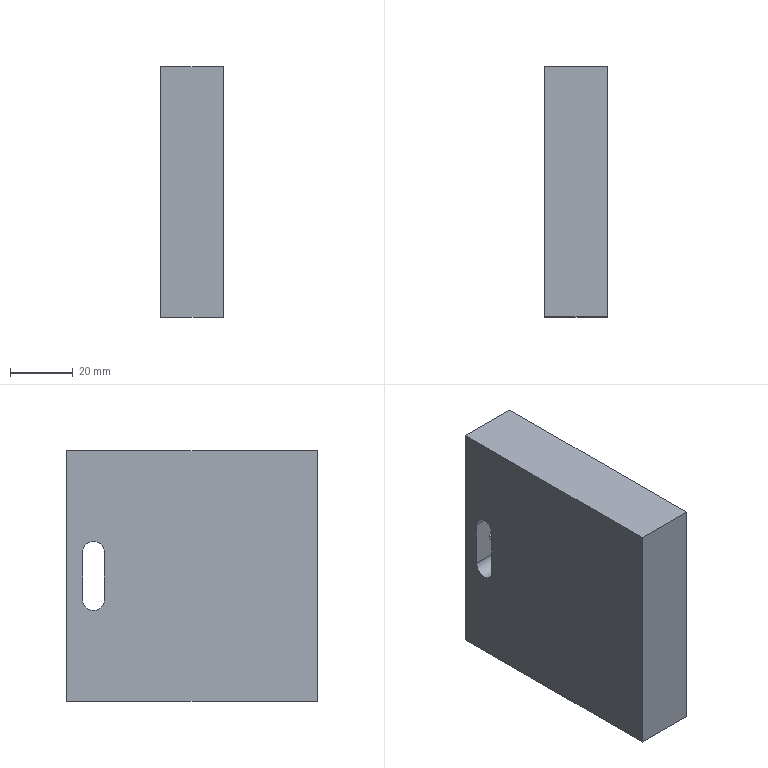Component | SolidWorks | LocatingDie-2_Die-1 | 1 solid | 14 faces | box 20 x 80 x 80 mm | volume 124605 mm3 | plane 10 | cylinder 4 | commonest cylinder face diameters 7 x3 8 x1
build123d program:
from build123d import *

# Parameters (mm, degrees)
SKETCH1_W      = 80
SKETCH1_H      = 80
EXTRUDE1_DEPTH = 20
EXTRUDE2_REACH = 95.62


with BuildPart() as part:
    # Sketch1 → Extrude1 (new body)
    with BuildSketch(Plane.XY):
        with Locations((-4.325, -1.62)):
            Rectangle(SKETCH1_W, SKETCH1_H)
        with BuildLine():
            Line((-11.825, 33.38), (3.175, 33.38))
            ThreePointArc((3.175, 33.38), (6.675, 29.88), (3.175, 26.38))
            Line((3.175, 26.38), (-11.825, 26.38))
            ThreePointArc((-11.825, 26.38), (-15.325, 29.88), (-11.825, 33.38))
        make_face(mode=Mode.SUBTRACT)
    extrude(amount=EXTRUDE1_DEPTH)

    # Sketch2 → Extrude2 (cut, up to next)
    with BuildSketch(Plane(origin=(0, 38.38, 0), x_dir=(1, 0, 0), z_dir=(0, 1, 0)), mode=Mode.PRIVATE) as extrude2_sk1:
        with BuildLine():
            Line((-0.3255, -20), (-8.325, -20))
            Line((-8.325, -20), (-8.325, -10))
            ThreePointArc((-8.325, -10), (-4.325, -6), (-0.3255, -10))
            Line((-0.3255, -10), (-0.3255, -20))
        make_face()
    extrude2_tool1 = extrude(extrude2_sk1.sketch, amount=-EXTRUDE2_REACH, mode=Mode.PRIVATE) & part.part
    add(extrude2_tool1.solids().sort_by_distance((-4.325, 38.38, 13.399))[0], mode=Mode.SUBTRACT)


solid = part.part

# Placed as in the assembly
solid = solid.moved(Location((-306.784, 563.808, 9.675), (0, 90, 0)))
STEP:
#1=COLOUR_RGB('',0.7922,0.8196,0.9333);
#2=FILL_AREA_STYLE_COLOUR('',#1);
#3=FILL_AREA_STYLE('',(#2));
#4=SURFACE_STYLE_FILL_AREA(#3);
#5=SURFACE_SIDE_STYLE('',(#4));
#6=SURFACE_STYLE_USAGE(.BOTH.,#5);
#7=PRESENTATION_STYLE_ASSIGNMENT((#6));
#8=CARTESIAN_POINT('',(-11.291,23.511,0.8465));
#9=VERTEX_POINT('',#8);
#10=CARTESIAN_POINT('',(-11.291,23.374,0.9843));
#11=VERTEX_POINT('',#10);
#12=CARTESIAN_POINT('',(-11.291,23.374,0.8465));
#13=DIRECTION('',(1.,0.,-0.));
#14=DIRECTION('',(-0.,0.,-1.));
#15=AXIS2_PLACEMENT_3D('',#12,#13,#14);
#16=CIRCLE('',#15,0.1378);
#17=EDGE_CURVE('',#9,#11,#16,.T.);
#18=ORIENTED_EDGE('',*,*,#17,.T.);
#19=CARTESIAN_POINT('',(-12.078,23.374,0.9843));
#20=VERTEX_POINT('',#19);
#21=CARTESIAN_POINT('',(-11.291,23.374,0.9843));
#22=DIRECTION('',(-1.,-0.,0.));
#23=VECTOR('',#22,39.37);
#24=LINE('',#21,#23);
#25=EDGE_CURVE('',#11,#20,#24,.T.);
#26=ORIENTED_EDGE('',*,*,#25,.T.);
#27=CARTESIAN_POINT('',(-12.078,23.511,0.8465));
#28=VERTEX_POINT('',#27);
#29=CARTESIAN_POINT('',(-12.078,23.374,0.8465));
#30=DIRECTION('',(1.,0.,-0.));
#31=DIRECTION('',(-0.,0.,-1.));
#32=AXIS2_PLACEMENT_3D('',#29,#30,#31);
#33=CIRCLE('',#32,0.1378);
#34=EDGE_CURVE('',#28,#20,#33,.T.);
#35=ORIENTED_EDGE('',*,*,#34,.F.);
#36=CARTESIAN_POINT('',(-11.291,23.511,0.8465));
#37=DIRECTION('',(-1.,-0.,0.));
#38=VECTOR('',#37,39.37);
#39=LINE('',#36,#38);
#40=EDGE_CURVE('',#9,#28,#39,.T.);
#41=ORIENTED_EDGE('',*,*,#40,.F.);
#42=EDGE_LOOP('',(#18,#26,#35,#41));
#43=FACE_OUTER_BOUND('',#42,.T.);
#44=CARTESIAN_POINT('',(-11.291,23.374,0.8465));
#45=DIRECTION('',(-1.,-0.,0.));
#46=DIRECTION('',(0.,0.,1.));
#47=AXIS2_PLACEMENT_3D('',#44,#45,#46);
#48=CYLINDRICAL_SURFACE('',#47,0.1378);
#49=ADVANCED_FACE('',(#43),#48,.F.);
#50=CARTESIAN_POINT('',(-11.291,23.511,0.7087));
#51=VERTEX_POINT('',#50);
#52=CARTESIAN_POINT('',(-11.291,23.708,0.7087));
#53=VERTEX_POINT('',#52);
#54=CARTESIAN_POINT('',(-11.291,20.559,0.7087));
#55=DIRECTION('',(-0.,1.,-0.));
#56=VECTOR('',#55,39.37);
#57=LINE('',#54,#56);
#58=EDGE_CURVE('',#51,#53,#57,.T.);
#59=ORIENTED_EDGE('',*,*,#58,.T.);
#60=CARTESIAN_POINT('',(-11.291,23.708,2.126));
#61=VERTEX_POINT('',#60);
#62=CARTESIAN_POINT('',(-11.291,23.708,2.126));
#63=DIRECTION('',(0.,0.,1.));
#64=VECTOR('',#63,39.37);
#65=LINE('',#62,#64);
#66=EDGE_CURVE('',#53,#61,#65,.T.);
#67=ORIENTED_EDGE('',*,*,#66,.T.);
#68=CARTESIAN_POINT('',(-11.291,20.559,2.126));
#69=VERTEX_POINT('',#68);
#70=CARTESIAN_POINT('',(-11.291,23.708,2.126));
#71=DIRECTION('',(0.,-1.,0.));
#72=VECTOR('',#71,39.37);
#73=LINE('',#70,#72);
#74=EDGE_CURVE('',#61,#69,#73,.T.);
#75=ORIENTED_EDGE('',*,*,#74,.T.);
#76=CARTESIAN_POINT('',(-11.291,20.559,-1.024));
#77=VERTEX_POINT('',#76);
#78=CARTESIAN_POINT('',(-11.291,20.559,2.126));
#79=DIRECTION('',(-0.,-0.,-1.));
#80=VECTOR('',#79,39.37);
#81=LINE('',#78,#80);
#82=EDGE_CURVE('',#69,#77,#81,.T.);
#83=ORIENTED_EDGE('',*,*,#82,.T.);
#84=CARTESIAN_POINT('',(-11.291,23.708,-1.024));
#85=VERTEX_POINT('',#84);
#86=CARTESIAN_POINT('',(-11.291,23.708,-1.024));
#87=DIRECTION('',(-0.,1.,-0.));
#88=VECTOR('',#87,39.37);
#89=LINE('',#86,#88);
#90=EDGE_CURVE('',#77,#85,#89,.T.);
#91=ORIENTED_EDGE('',*,*,#90,.T.);
#92=CARTESIAN_POINT('',(-11.291,23.708,0.3937));
#93=VERTEX_POINT('',#92);
#94=CARTESIAN_POINT('',(-11.291,23.708,2.126));
#95=DIRECTION('',(0.,0.,1.));
#96=VECTOR('',#95,39.37);
#97=LINE('',#94,#96);
#98=EDGE_CURVE('',#85,#93,#97,.T.);
#99=ORIENTED_EDGE('',*,*,#98,.T.);
#100=CARTESIAN_POINT('',(-11.291,23.511,0.3937));
#101=VERTEX_POINT('',#100);
#102=CARTESIAN_POINT('',(-11.291,20.559,0.3937));
#103=DIRECTION('',(-0.,1.,-0.));
#104=VECTOR('',#103,39.37);
#105=LINE('',#102,#104);
#106=EDGE_CURVE('',#101,#93,#105,.T.);
#107=ORIENTED_EDGE('',*,*,#106,.F.);
#108=CARTESIAN_POINT('',(-11.291,23.511,0.2559));
#109=VERTEX_POINT('',#108);
#110=CARTESIAN_POINT('',(-11.291,23.511,0.8465));
#111=DIRECTION('',(0.,0.,1.));
#112=VECTOR('',#111,39.37);
#113=LINE('',#110,#112);
#114=EDGE_CURVE('',#109,#101,#113,.T.);
#115=ORIENTED_EDGE('',*,*,#114,.F.);
#116=CARTESIAN_POINT('',(-11.291,23.236,0.2559));
#117=VERTEX_POINT('',#116);
#118=CARTESIAN_POINT('',(-11.291,23.374,0.2559));
#119=DIRECTION('',(1.,0.,-0.));
#120=DIRECTION('',(-0.,0.,-1.));
#121=AXIS2_PLACEMENT_3D('',#118,#119,#120);
#122=CIRCLE('',#121,0.1378);
#123=EDGE_CURVE('',#117,#109,#122,.T.);
#124=ORIENTED_EDGE('',*,*,#123,.F.);
#125=CARTESIAN_POINT('',(-11.291,23.236,0.8465));
#126=VERTEX_POINT('',#125);
#127=CARTESIAN_POINT('',(-11.291,23.236,0.8465));
#128=DIRECTION('',(-0.,-0.,-1.));
#129=VECTOR('',#128,39.37);
#130=LINE('',#127,#129);
#131=EDGE_CURVE('',#126,#117,#130,.T.);
#132=ORIENTED_EDGE('',*,*,#131,.F.);
#133=CARTESIAN_POINT('',(-11.291,23.374,0.8465));
#134=DIRECTION('',(1.,0.,-0.));
#135=DIRECTION('',(-0.,0.,-1.));
#136=AXIS2_PLACEMENT_3D('',#133,#134,#135);
#137=CIRCLE('',#136,0.1378);
#138=EDGE_CURVE('',#11,#126,#137,.T.);
#139=ORIENTED_EDGE('',*,*,#138,.F.);
#140=ORIENTED_EDGE('',*,*,#17,.F.);
#141=CARTESIAN_POINT('',(-11.291,23.511,0.8465));
#142=DIRECTION('',(0.,0.,1.));
#143=VECTOR('',#142,39.37);
#144=LINE('',#141,#143);
#145=EDGE_CURVE('',#51,#9,#144,.T.);
#146=ORIENTED_EDGE('',*,*,#145,.F.);
#147=EDGE_LOOP('',(#59,#67,#75,#83,#91,#99,#107,#115,#124,#132,#139,#140,#146));
#148=FACE_OUTER_BOUND('',#147,.T.);
#149=CARTESIAN_POINT('',(-11.291,20.559,2.126));
#150=DIRECTION('',(1.,0.,-0.));
#151=DIRECTION('',(-0.,-0.,-1.));
#152=AXIS2_PLACEMENT_3D('',#149,#150,#151);
#153=PLANE('',#152);
#154=ADVANCED_FACE('',(#148),#153,.T.);
#155=CARTESIAN_POINT('',(-12.078,23.708,2.126));
#156=VERTEX_POINT('',#155);
#157=CARTESIAN_POINT('',(-12.078,20.559,2.126));
#158=VERTEX_POINT('',#157);
#159=CARTESIAN_POINT('',(-12.078,23.708,2.126));
#160=DIRECTION('',(0.,-1.,0.));
#161=VECTOR('',#160,39.37);
#162=LINE('',#159,#161);
#163=EDGE_CURVE('',#156,#158,#162,.T.);
#164=ORIENTED_EDGE('',*,*,#163,.F.);
#165=CARTESIAN_POINT('',(-12.078,23.708,-1.024));
#166=VERTEX_POINT('',#165);
#167=CARTESIAN_POINT('',(-12.078,23.708,2.126));
#168=DIRECTION('',(0.,0.,1.));
#169=VECTOR('',#168,39.37);
#170=LINE('',#167,#169);
#171=EDGE_CURVE('',#166,#156,#170,.T.);
#172=ORIENTED_EDGE('',*,*,#171,.F.);
#173=CARTESIAN_POINT('',(-12.078,20.559,-1.024));
#174=VERTEX_POINT('',#173);
#175=CARTESIAN_POINT('',(-12.078,23.708,-1.024));
#176=DIRECTION('',(-0.,1.,-0.));
#177=VECTOR('',#176,39.37);
#178=LINE('',#175,#177);
#179=EDGE_CURVE('',#174,#166,#178,.T.);
#180=ORIENTED_EDGE('',*,*,#179,.F.);
#181=CARTESIAN_POINT('',(-12.078,20.559,2.126));
#182=DIRECTION('',(-0.,-0.,-1.));
#183=VECTOR('',#182,39.37);
#184=LINE('',#181,#183);
#185=EDGE_CURVE('',#158,#174,#184,.T.);
#186=ORIENTED_EDGE('',*,*,#185,.F.);
#187=EDGE_LOOP('',(#164,#172,#180,#186));
#188=FACE_OUTER_BOUND('',#187,.T.);
#189=ORIENTED_EDGE('',*,*,#34,.T.);
#190=CARTESIAN_POINT('',(-12.078,23.236,0.8465));
#191=VERTEX_POINT('',#190);
#192=CARTESIAN_POINT('',(-12.078,23.374,0.8465));
#193=DIRECTION('',(1.,0.,-0.));
#194=DIRECTION('',(-0.,0.,-1.));
#195=AXIS2_PLACEMENT_3D('',#192,#193,#194);
#196=CIRCLE('',#195,0.1378);
#197=EDGE_CURVE('',#20,#191,#196,.T.);
#198=ORIENTED_EDGE('',*,*,#197,.T.);
#199=CARTESIAN_POINT('',(-12.078,23.236,0.2559));
#200=VERTEX_POINT('',#199);
#201=CARTESIAN_POINT('',(-12.078,23.236,0.8465));
#202=DIRECTION('',(-0.,-0.,-1.));
#203=VECTOR('',#202,39.37);
#204=LINE('',#201,#203);
#205=EDGE_CURVE('',#191,#200,#204,.T.);
#206=ORIENTED_EDGE('',*,*,#205,.T.);
#207=CARTESIAN_POINT('',(-12.078,23.511,0.2559));
#208=VERTEX_POINT('',#207);
#209=CARTESIAN_POINT('',(-12.078,23.374,0.2559));
#210=DIRECTION('',(1.,0.,-0.));
#211=DIRECTION('',(-0.,0.,-1.));
#212=AXIS2_PLACEMENT_3D('',#209,#210,#211);
#213=CIRCLE('',#212,0.1378);
#214=EDGE_CURVE('',#200,#208,#213,.T.);
#215=ORIENTED_EDGE('',*,*,#214,.T.);
#216=CARTESIAN_POINT('',(-12.078,23.511,0.8465));
#217=DIRECTION('',(0.,0.,1.));
#218=VECTOR('',#217,39.37);
#219=LINE('',#216,#218);
#220=EDGE_CURVE('',#208,#28,#219,.T.);
#221=ORIENTED_EDGE('',*,*,#220,.T.);
#222=EDGE_LOOP('',(#189,#198,#206,#215,#221));
#223=FACE_BOUND('',#222,.T.);
#224=CARTESIAN_POINT('',(-12.078,20.559,2.126));
#225=DIRECTION('',(1.,0.,-0.));
#226=DIRECTION('',(-0.,-0.,-1.));
#227=AXIS2_PLACEMENT_3D('',#224,#225,#226);
#228=PLANE('',#227);
#229=ADVANCED_FACE('',(#188,#223),#228,.F.);
#230=ORIENTED_EDGE('',*,*,#163,.T.);
#231=CARTESIAN_POINT('',(-11.291,20.559,2.126));
#232=DIRECTION('',(-1.,-0.,0.));
#233=VECTOR('',#232,39.37);
#234=LINE('',#231,#233);
#235=EDGE_CURVE('',#69,#158,#234,.T.);
#236=ORIENTED_EDGE('',*,*,#235,.F.);
#237=ORIENTED_EDGE('',*,*,#74,.F.);
#238=CARTESIAN_POINT('',(-11.291,23.708,2.126));
#239=DIRECTION('',(-1.,-0.,0.));
#240=VECTOR('',#239,39.37);
#241=LINE('',#238,#240);
#242=EDGE_CURVE('',#61,#156,#241,.T.);
#243=ORIENTED_EDGE('',*,*,#242,.T.);
#244=EDGE_LOOP('',(#230,#236,#237,#243));
#245=FACE_OUTER_BOUND('',#244,.T.);
#246=CARTESIAN_POINT('',(-11.291,23.708,2.126));
#247=DIRECTION('',(-0.,-0.,-1.));
#248=DIRECTION('',(-0.,1.,-0.));
#249=AXIS2_PLACEMENT_3D('',#246,#247,#248);
#250=PLANE('',#249);
#251=ADVANCED_FACE('',(#245),#250,.F.);
#252=ORIENTED_EDGE('',*,*,#185,.T.);
#253=CARTESIAN_POINT('',(-11.291,20.559,-1.024));
#254=DIRECTION('',(-1.,-0.,0.));
#255=VECTOR('',#254,39.37);
#256=LINE('',#253,#255);
#257=EDGE_CURVE('',#77,#174,#256,.T.);
#258=ORIENTED_EDGE('',*,*,#257,.F.);
#259=ORIENTED_EDGE('',*,*,#82,.F.);
#260=ORIENTED_EDGE('',*,*,#235,.T.);
#261=EDGE_LOOP('',(#252,#258,#259,#260));
#262=FACE_OUTER_BOUND('',#261,.T.);
#263=CARTESIAN_POINT('',(-11.291,20.559,2.126));
#264=DIRECTION('',(-0.,1.,-0.));
#265=DIRECTION('',(0.,0.,1.));
#266=AXIS2_PLACEMENT_3D('',#263,#264,#265);
#267=PLANE('',#266);
#268=ADVANCED_FACE('',(#262),#267,.F.);
#269=ORIENTED_EDGE('',*,*,#179,.T.);
#270=CARTESIAN_POINT('',(-11.291,23.708,-1.024));
#271=DIRECTION('',(-1.,-0.,0.));
#272=VECTOR('',#271,39.37);
#273=LINE('',#270,#272);
#274=EDGE_CURVE('',#85,#166,#273,.T.);
#275=ORIENTED_EDGE('',*,*,#274,.F.);
#276=ORIENTED_EDGE('',*,*,#90,.F.);
#277=ORIENTED_EDGE('',*,*,#257,.T.);
#278=EDGE_LOOP('',(#269,#275,#276,#277));
#279=FACE_OUTER_BOUND('',#278,.T.);
#280=CARTESIAN_POINT('',(-11.291,23.708,-1.024));
#281=DIRECTION('',(0.,0.,1.));
#282=DIRECTION('',(0.,-1.,0.));
#283=AXIS2_PLACEMENT_3D('',#280,#281,#282);
#284=PLANE('',#283);
#285=ADVANCED_FACE('',(#279),#284,.F.);
#286=ORIENTED_EDGE('',*,*,#66,.F.);
#287=CARTESIAN_POINT('',(-11.684,23.708,0.7087));
#288=VERTEX_POINT('',#287);
#289=CARTESIAN_POINT('',(-11.291,23.708,0.7087));
#290=DIRECTION('',(1.,0.,-0.));
#291=VECTOR('',#290,39.37);
#292=LINE('',#289,#291);
#293=EDGE_CURVE('',#288,#53,#292,.T.);
#294=ORIENTED_EDGE('',*,*,#293,.F.);
#295=CARTESIAN_POINT('',(-11.684,23.708,0.3937));
#296=VERTEX_POINT('',#295);
#297=CARTESIAN_POINT('',(-11.684,23.708,0.5512));
#298=DIRECTION('',(-0.,1.,-0.));
#299=DIRECTION('',(0.,0.,1.));
#300=AXIS2_PLACEMENT_3D('',#297,#298,#299);
#301=CIRCLE('',#300,0.1575);
#302=EDGE_CURVE('',#296,#288,#301,.T.);
#303=ORIENTED_EDGE('',*,*,#302,.F.);
#304=CARTESIAN_POINT('',(-11.291,23.708,0.3937));
#305=DIRECTION('',(-1.,-0.,0.));
#306=VECTOR('',#305,39.37);
#307=LINE('',#304,#306);
#308=EDGE_CURVE('',#93,#296,#307,.T.);
#309=ORIENTED_EDGE('',*,*,#308,.F.);
#310=ORIENTED_EDGE('',*,*,#98,.F.);
#311=ORIENTED_EDGE('',*,*,#274,.T.);
#312=ORIENTED_EDGE('',*,*,#171,.T.);
#313=ORIENTED_EDGE('',*,*,#242,.F.);
#314=EDGE_LOOP('',(#286,#294,#303,#309,#310,#311,#312,#313));
#315=FACE_OUTER_BOUND('',#314,.T.);
#316=CARTESIAN_POINT('',(-11.291,23.708,2.126));
#317=DIRECTION('',(0.,-1.,0.));
#318=DIRECTION('',(-0.,-0.,-1.));
#319=AXIS2_PLACEMENT_3D('',#316,#317,#318);
#320=PLANE('',#319);
#321=ADVANCED_FACE('',(#315),#320,.F.);
#322=ORIENTED_EDGE('',*,*,#25,.F.);
#323=ORIENTED_EDGE('',*,*,#138,.T.);
#324=CARTESIAN_POINT('',(-11.291,23.236,0.8465));
#325=DIRECTION('',(-1.,-0.,0.));
#326=VECTOR('',#325,39.37);
#327=LINE('',#324,#326);
#328=EDGE_CURVE('',#126,#191,#327,.T.);
#329=ORIENTED_EDGE('',*,*,#328,.T.);
#330=ORIENTED_EDGE('',*,*,#197,.F.);
#331=EDGE_LOOP('',(#322,#323,#329,#330));
#332=FACE_OUTER_BOUND('',#331,.T.);
#333=CARTESIAN_POINT('',(-11.291,23.374,0.8465));
#334=DIRECTION('',(-1.,-0.,0.));
#335=DIRECTION('',(0.,0.,1.));
#336=AXIS2_PLACEMENT_3D('',#333,#334,#335);
#337=CYLINDRICAL_SURFACE('',#336,0.1378);
#338=ADVANCED_FACE('',(#332),#337,.F.);
#339=ORIENTED_EDGE('',*,*,#205,.F.);
#340=ORIENTED_EDGE('',*,*,#328,.F.);
#341=ORIENTED_EDGE('',*,*,#131,.T.);
#342=CARTESIAN_POINT('',(-11.291,23.236,0.2559));
#343=DIRECTION('',(-1.,-0.,0.));
#344=VECTOR('',#343,39.37);
#345=LINE('',#342,#344);
#346=EDGE_CURVE('',#117,#200,#345,.T.);
#347=ORIENTED_EDGE('',*,*,#346,.T.);
#348=EDGE_LOOP('',(#339,#340,#341,#347));
#349=FACE_OUTER_BOUND('',#348,.T.);
#350=CARTESIAN_POINT('',(-11.291,23.236,0.8465));
#351=DIRECTION('',(-0.,1.,-0.));
#352=DIRECTION('',(1.,0.,-0.));
#353=AXIS2_PLACEMENT_3D('',#350,#351,#352);
#354=PLANE('',#353);
#355=ADVANCED_FACE('',(#349),#354,.T.);
#356=ORIENTED_EDGE('',*,*,#214,.F.);
#357=ORIENTED_EDGE('',*,*,#346,.F.);
#358=ORIENTED_EDGE('',*,*,#123,.T.);
#359=CARTESIAN_POINT('',(-11.291,23.511,0.2559));
#360=DIRECTION('',(-1.,-0.,0.));
#361=VECTOR('',#360,39.37);
#362=LINE('',#359,#361);
#363=EDGE_CURVE('',#109,#208,#362,.T.);
#364=ORIENTED_EDGE('',*,*,#363,.T.);
#365=EDGE_LOOP('',(#356,#357,#358,#364));
#366=FACE_OUTER_BOUND('',#365,.T.);
#367=CARTESIAN_POINT('',(-11.291,23.374,0.2559));
#368=DIRECTION('',(-1.,-0.,0.));
#369=DIRECTION('',(0.,0.,1.));
#370=AXIS2_PLACEMENT_3D('',#367,#368,#369);
#371=CYLINDRICAL_SURFACE('',#370,0.1378);
#372=ADVANCED_FACE('',(#366),#371,.F.);
#373=CARTESIAN_POINT('',(-11.684,23.511,0.7087));
#374=VERTEX_POINT('',#373);
#375=CARTESIAN_POINT('',(-11.291,23.511,0.7087));
#376=DIRECTION('',(1.,0.,-0.));
#377=VECTOR('',#376,39.37);
#378=LINE('',#375,#377);
#379=EDGE_CURVE('',#374,#51,#378,.T.);
#380=ORIENTED_EDGE('',*,*,#379,.T.);
#381=ORIENTED_EDGE('',*,*,#145,.T.);
#382=ORIENTED_EDGE('',*,*,#40,.T.);
#383=ORIENTED_EDGE('',*,*,#220,.F.);
#384=ORIENTED_EDGE('',*,*,#363,.F.);
#385=ORIENTED_EDGE('',*,*,#114,.T.);
#386=CARTESIAN_POINT('',(-11.684,23.511,0.3937));
#387=VERTEX_POINT('',#386);
#388=CARTESIAN_POINT('',(-11.291,23.511,0.3937));
#389=DIRECTION('',(-1.,-0.,0.));
#390=VECTOR('',#389,39.37);
#391=LINE('',#388,#390);
#392=EDGE_CURVE('',#101,#387,#391,.T.);
#393=ORIENTED_EDGE('',*,*,#392,.T.);
#394=CARTESIAN_POINT('',(-11.684,23.511,0.5512));
#395=DIRECTION('',(-0.,1.,-0.));
#396=DIRECTION('',(-1.,0.,0.));
#397=AXIS2_PLACEMENT_3D('',#394,#395,#396);
#398=CIRCLE('',#397,0.1575);
#399=EDGE_CURVE('',#387,#374,#398,.T.);
#400=ORIENTED_EDGE('',*,*,#399,.T.);
#401=EDGE_LOOP('',(#380,#381,#382,#383,#384,#385,#393,#400));
#402=FACE_OUTER_BOUND('',#401,.T.);
#403=CARTESIAN_POINT('',(-11.291,23.511,0.8465));
#404=DIRECTION('',(0.,-1.,0.));
#405=DIRECTION('',(-1.,-0.,0.));
#406=AXIS2_PLACEMENT_3D('',#403,#404,#405);
#407=PLANE('',#406);
#408=ADVANCED_FACE('',(#402),#407,.T.);
#409=CARTESIAN_POINT('',(-11.684,20.559,0.3937));
#410=DIRECTION('',(-0.,1.,-0.));
#411=VECTOR('',#410,39.37);
#412=LINE('',#409,#411);
#413=EDGE_CURVE('',#387,#296,#412,.T.);
#414=ORIENTED_EDGE('',*,*,#413,.T.);
#415=ORIENTED_EDGE('',*,*,#302,.T.);
#416=CARTESIAN_POINT('',(-11.684,20.559,0.7087));
#417=DIRECTION('',(-0.,1.,-0.));
#418=VECTOR('',#417,39.37);
#419=LINE('',#416,#418);
#420=EDGE_CURVE('',#374,#288,#419,.T.);
#421=ORIENTED_EDGE('',*,*,#420,.F.);
#422=ORIENTED_EDGE('',*,*,#399,.F.);
#423=EDGE_LOOP('',(#414,#415,#421,#422));
#424=FACE_OUTER_BOUND('',#423,.T.);
#425=CARTESIAN_POINT('',(-11.684,20.559,0.5512));
#426=DIRECTION('',(-0.,1.,-0.));
#427=DIRECTION('',(0.,0.,1.));
#428=AXIS2_PLACEMENT_3D('',#425,#426,#427);
#429=CYLINDRICAL_SURFACE('',#428,0.1575);
#430=ADVANCED_FACE('',(#424),#429,.F.);
#431=ORIENTED_EDGE('',*,*,#420,.T.);
#432=ORIENTED_EDGE('',*,*,#293,.T.);
#433=ORIENTED_EDGE('',*,*,#58,.F.);
#434=ORIENTED_EDGE('',*,*,#379,.F.);
#435=EDGE_LOOP('',(#431,#432,#433,#434));
#436=FACE_OUTER_BOUND('',#435,.T.);
#437=CARTESIAN_POINT('',(-11.291,20.559,0.7087));
#438=DIRECTION('',(0.,0.,1.));
#439=DIRECTION('',(1.,0.,-0.));
#440=AXIS2_PLACEMENT_3D('',#437,#438,#439);
#441=PLANE('',#440);
#442=ADVANCED_FACE('',(#436),#441,.F.);
#443=ORIENTED_EDGE('',*,*,#106,.T.);
#444=ORIENTED_EDGE('',*,*,#308,.T.);
#445=ORIENTED_EDGE('',*,*,#413,.F.);
#446=ORIENTED_EDGE('',*,*,#392,.F.);
#447=EDGE_LOOP('',(#443,#444,#445,#446));
#448=FACE_OUTER_BOUND('',#447,.T.);
#449=CARTESIAN_POINT('',(-11.291,20.559,0.3937));
#450=DIRECTION('',(-0.,-0.,-1.));
#451=DIRECTION('',(-0.,1.,-0.));
#452=AXIS2_PLACEMENT_3D('',#449,#450,#451);
#453=PLANE('',#452);
#454=ADVANCED_FACE('',(#448),#453,.F.);
#455=CLOSED_SHELL('',(#49,#154,#229,#251,#268,#285,#321,#338,#355,#372,#408,#430,#442,#454));
#456=MANIFOLD_SOLID_BREP('',#455);
#457=STYLED_ITEM('',(#7),#456);
#458=PRESENTATION_LAYER_ASSIGNMENT('','',(#457));
#459=(LENGTH_UNIT()NAMED_UNIT(*)SI_UNIT($,.METRE.));
#460=LENGTH_MEASURE_WITH_UNIT(LENGTH_MEASURE(0.0254),#459);
#461=DIMENSIONAL_EXPONENTS(1.,0.,0.,0.,0.,0.,0.);
#462=(CONVERSION_BASED_UNIT('',#460)LENGTH_UNIT()NAMED_UNIT(#461));
#463=UNCERTAINTY_MEASURE_WITH_UNIT(LENGTH_MEASURE(0.00001),#462,'','');
#464=(NAMED_UNIT(*)PLANE_ANGLE_UNIT()SI_UNIT($,.RADIAN.));
#465=(NAMED_UNIT(*)SI_UNIT($,.STERADIAN.)SOLID_ANGLE_UNIT());
#466=(GEOMETRIC_REPRESENTATION_CONTEXT(3)GLOBAL_UNCERTAINTY_ASSIGNED_CONTEXT((#463))GLOBAL_UNIT_ASSIGNED_CONTEXT((#462,#464,#465))REPRESENTATION_CONTEXT('',''));
#467=MECHANICAL_DESIGN_GEOMETRIC_PRESENTATION_REPRESENTATION('',(#457),#466);
#468=CARTESIAN_POINT('',(0.,0.,0.));
#469=DIRECTION('',(0.,0.,1.));
#470=DIRECTION('',(1.,0.,0.));
#471=AXIS2_PLACEMENT_3D('',#468,#469,#470);
#472=(LENGTH_UNIT()NAMED_UNIT(*)SI_UNIT($,.METRE.));
#473=LENGTH_MEASURE_WITH_UNIT(LENGTH_MEASURE(0.0254),#472);
#474=DIMENSIONAL_EXPONENTS(1.,0.,0.,0.,0.,0.,0.);
#475=(CONVERSION_BASED_UNIT('',#473)LENGTH_UNIT()NAMED_UNIT(#474));
#476=UNCERTAINTY_MEASURE_WITH_UNIT(LENGTH_MEASURE(0.00001),#475,'','');
#477=(NAMED_UNIT(*)PLANE_ANGLE_UNIT()SI_UNIT($,.RADIAN.));
#478=(NAMED_UNIT(*)SI_UNIT($,.STERADIAN.)SOLID_ANGLE_UNIT());
#479=(GEOMETRIC_REPRESENTATION_CONTEXT(3)GLOBAL_UNCERTAINTY_ASSIGNED_CONTEXT((#476))GLOBAL_UNIT_ASSIGNED_CONTEXT((#475,#477,#478))REPRESENTATION_CONTEXT('',''));
#480=ADVANCED_BREP_SHAPE_REPRESENTATION('',(#456,#471),#479);